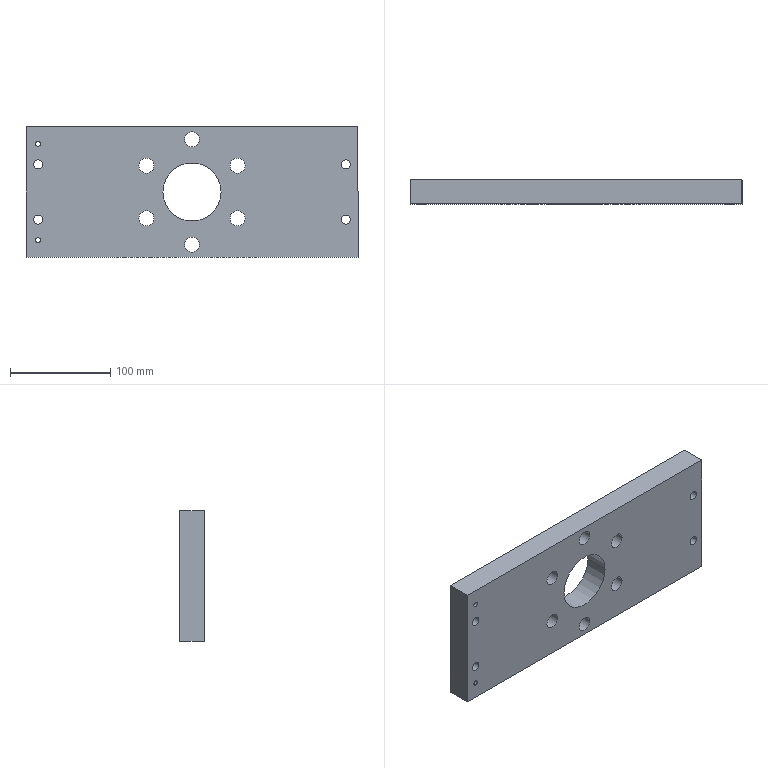Component | SolidWorks | DrillTemplate-1 | 1 solid | 86 faces | box 331 x 24 x 130 mm | volume 929794 mm3 | cylinder 58 | plane 16 | cone 12 | commonest cylinder face diameters 15 x20 6 x12 10 x12 9 x8 5 x4 58 x2
build123d program:
from build123d import *

# Parameters (mm, degrees)
SKETCH1_2_W                                          = 331
SKETCH1_2_H                                          = 130
BOSS_EXTRUDE1_DEPTH                                  = 24
SKETCH2_R                                            = 29
CUT_EXTRUDE1_DEPTH                                   = 64
CIRPATTERN1_COUNT                                    = 6
CIRPATTERN2_COUNT                                    = 6
SIZE_MM_DOWEL_PIN_HOLE_1_D                           = 5
HOLE_SIZE_ACCORDING_TO_HEXAGON_SOCKET_HE_D           = 9
HOLE_SIZE_ACCORDING_TO_HEXAGON_SOCKET_HE_CBORE_D     = 15
HOLE_SIZE_ACCORDING_TO_HEXAGON_SOCKET_HE_CBORE_DEPTH = 9
SKETCH1_R                                            = 5
BUSHINGSCREWCOLLARRELIEF_DEPTH                       = 1


with BuildPart() as part:
    # Sketch1_2 → Boss-Extrude1 (new body)
    with BuildSketch(Plane.XY):
        Rectangle(SKETCH1_2_W, SKETCH1_2_H)
    extrude(amount=-BOSS_EXTRUDE1_DEPTH)

    # Sketch2 → Cut-Extrude1 (cut)
    with BuildSketch(Plane.XY):
        Circle(SKETCH2_R)
    extrude(amount=-CUT_EXTRUDE1_DEPTH, mode=Mode.SUBTRACT)

    # Sketch4 → 15.0 _15_ Diameter Hole1 (revolve, cut)
    with BuildSketch(Plane(origin=(0, -52.5, 0), x_dir=(0, -1, 0), z_dir=(1, 0, 0))):
        Polygon((0, 0), (0, 33.33), (7.5, 29), (7.5, 0), align=None)
    f_15_0_15_diameter_hole1 = revolve(axis=Axis((0, -52.5, 6.35), (0, 0, -1)), mode=Mode.SUBTRACT)

    # CirPattern1: 15.0 _15_ Diameter Hole1 ×6 about axis
    cirpattern1_axis = Axis((0, 0, 0), (0, 0, 1))
    for i in range(1, CIRPATTERN1_COUNT):
        add(f_15_0_15_diameter_hole1.rotate(cirpattern1_axis, i * 360 / CIRPATTERN1_COUNT), mode=Mode.SUBTRACT)

    # Sketch6 → M6x1.0 Tapped Hole1 (revolve, cut)
    with BuildSketch(Plane(origin=(0, -37.5, 0), x_dir=(0, -1, 0), z_dir=(1, 0, 0))):
        Polygon((0, 0), (0, 16.803), (3, 15), (3, 0), align=None)
    m6x1_0_tapped_hole1 = revolve(axis=Axis((0, -37.5, 6.35), (0, 0, -1)), mode=Mode.SUBTRACT)

    # CirPattern2: M6x1.0 Tapped Hole1 ×6 about axis
    cirpattern2_axis = Axis((0, 0, 0), (0, 0, 1))
    for i in range(1, CIRPATTERN2_COUNT):
        add(m6x1_0_tapped_hole1.rotate(cirpattern2_axis, i * 360 / CIRPATTERN2_COUNT), mode=Mode.SUBTRACT)

    # Size mm Dowel Pin Hole 1 (through all)
    with Locations(Plane.XY):
        with Locations((-153.5, 48), (-153.5, -48)):
            Hole(SIZE_MM_DOWEL_PIN_HOLE_1_D / 2)

    # Hole Size_According to_Hexagon Socket He (through all)
    with Locations(Plane.XY):
        with Locations((-153.5, 27.5), (-153.5, -27.5)):
            hole_size_according_to_hexagon_socket_he = CounterBoreHole(HOLE_SIZE_ACCORDING_TO_HEXAGON_SOCKET_HE_D / 2, HOLE_SIZE_ACCORDING_TO_HEXAGON_SOCKET_HE_CBORE_D / 2, HOLE_SIZE_ACCORDING_TO_HEXAGON_SOCKET_HE_CBORE_DEPTH)

    # Mirror1: Hole Size_According to_Hexagon Socket He across plane
    add(hole_size_according_to_hexagon_socket_he.mirror(Plane(origin=(0, 0, 0), x_dir=(0, 0, 1), z_dir=(1, 0, 0))), mode=Mode.SUBTRACT)

    # Sketch1 → BushingScrewCollarRelief (cut)
    with BuildSketch(Plane.XY):
        with Locations((0, 37.5)):
            Circle(SKETCH1_R)
        with Locations((0, -37.5)):
            Circle(SKETCH1_R)
        with Locations((32.476, 18.75)):
            Circle(SKETCH1_R)
        with Locations((32.476, -18.75)):
            Circle(SKETCH1_R)
        with Locations((-32.476, 18.75)):
            Circle(SKETCH1_R)
        with Locations((-32.476, -18.75)):
            Circle(SKETCH1_R)
    extrude(amount=-BUSHINGSCREWCOLLARRELIEF_DEPTH, mode=Mode.SUBTRACT)


solid = part.part

# Placed as in the assembly
solid = solid.moved(Location((0, 305, 0), (-90, 0, 0)))